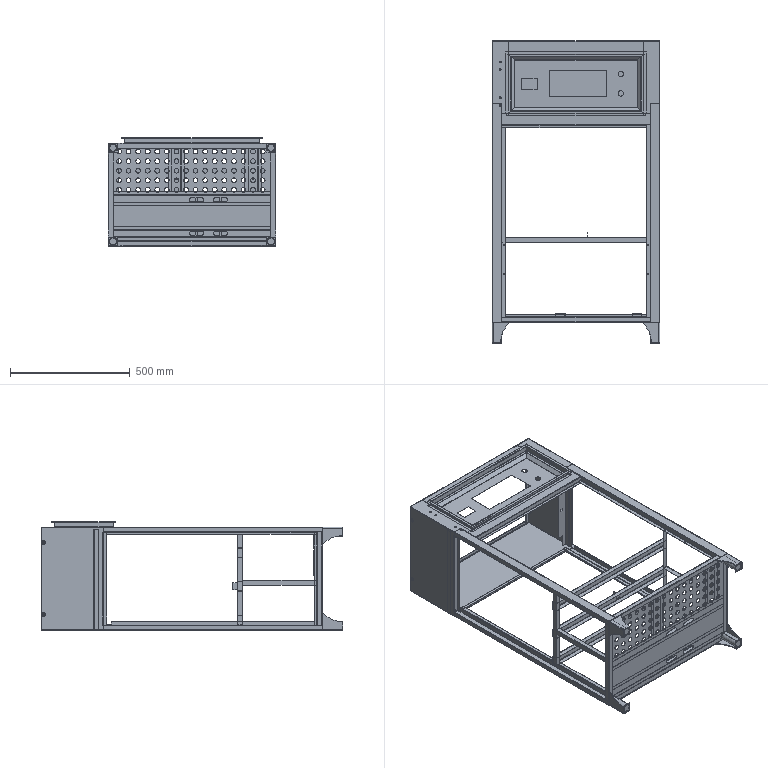Assembly | SolidWorks | mm | 51 component files | 51 solids | 1512 faces | box 700 x 1261 x 452 mm | volume 2289433 mm3 | plane 968 | cylinder 496 | cone 32 | spline 16 | commonest cylinder face diameters 20 x160 1.473 x95 3.473 x91 5 x48 6 x30 18 x12 10 x12 8 x8
Bill of materials:
12x1x12WeldedSquare | 4 | 304 | Thin, flat, square plate with no visible holes or other features.
CCQ-1.1-10Panel | 1 | 304 | Shallow rectangular tray or recessed panel. It has a flat floor, angled walls on all four sides, and a thin flat rim around the outside. The floor has one small rectangular cutout, one large rectangular cutout, and two small round holes.
CCQ-1.1-11UpperBeam1 | 1 | 304 | Long, thin-wall bent profile with a stepped, hat-like cross-section and rounded bends. In section it runs: bottom flange, vertical wall, raised horizontal wall, second vertical wall, short top return lip. One small round hole is near one end.
CCQ-1.1-12LowerBeam2 | 2 | 304 | Short, straight, thin-wall bent profile with three rounded bends. In section it runs: short leg, horizontal wall, long wall, horizontal wall. There is one small round hole near each end on one face.
CCQ-1.1-13UpperBeam2 | 1 | 304 | Long, thin-wall bent channel with three rounded bends. In section it has a short top lip, a vertical wall, a wide base, and a downward leg at the far edge. No holes are visible.
CCQ-1.1-14LowerSidePost1 | 2 | 304 | Long, thin-wall bent profile with five rounded bends. In section it forms a box-like channel with an outward flange on one side and an upward return lip on the other. No holes are visible.
CCQ-1.1-15LowerSidePost2 | 1 | 304 | Long, thin-wall bent profile with five rounded bends. In section it forms a near-closed box shape with two legs leaving in opposite directions (one horizontal flange, one vertical leg). There are small holes along one flange.
CCQ-1.1-16LowerSidePost3 | 1 | 304 | Long, thin-wall bent profile with five rounded bends. In section it forms a near-closed box shape with a downward leg and a horizontal outward flange. There is one round hole near one end on the top face and small holes along a flange. One flange is cut back near one end.
CCQ-1.1-17LowerBeam1 | 2 | 304 | Long bent profile with three rounded bends. In section it is an inverted U (channel) with an outward horizontal flange on one leg. The wall looks thicker relative to the section size than on the other profiles. No holes are visible.
CCQ-1.1-18Limiter | 1 | 304 | Short L-shaped angle with legs of about equal length and a single rounded bend. No holes are visible.
CCQ-1.1-19Support1 | 2 | 304 | Straight hat-section (omega-shaped) profile. It has a raised flat top, two vertical walls, and two outward flanges at the base, with rounded bends. There are two small round holes on the raised top face.
CCQ-1.1-1AngleIron | 2 | 304 | Long, slender L-shaped angle with legs of about equal length and a single rounded bend. No holes are visible.
CCQ-1.1-20Support2 | 2 | 304 | Long, straight hat-section (omega) profile made of thin formed sheet: a central U-shaped channel with two outward flanges, plus two obround slots through the channel floor.
CCQ-1.1-21SupportBendPart | 4 | 304 | Short thin angle piece with two legs at 90 degrees joined by a rounded bend. Each leg has a large concave curved cutout on its free edge, so the legs taper toward the bend corner.
CCQ-1.1-22VerticalAngleIron | 2 | 304 | Long, straight, plain L-angle profile of thin wall with a rounded inside bend and roughly equal legs.
CCQ-1.1-23BendPart | 3 | 304 | Long, straight C/U channel profile with a flat web, two parallel flanges and rounded bends. Two small round holes sit close together in the web near one end.
CCQ-1.1-2UpperAngleIron | 2 | 304 | Straight L-angle profile with unequal leg treatment: one leg runs the full length, while the other leg covers only a central portion, with stepped cutbacks at both ends. That partial leg has two elongated slots.
CCQ-1.1-3SideUpperPlate2 | 2 | 304 | Large, flat, rectangular thin sheet panel with formed edges. One long edge has a short return flange. The opposite edge has a flange with a small offset/downturned lip (joggle-like step). There are two small round holes near one side and a narrower, shorter flange strip along the other side.
CCQ-1.1-4SideUpperPlate1 | 1 | 304 | Rectangular, flat thin sheet panel with short upturned flanges along both long edges. One edge has an outward offset step before its lip. Small holes are visible near the flange ends.
CCQ-1.1-5SideUpperPlate3 | 1 | 304 | Elongated formed sheet bracket. A flat base plate joins a vertical wall that ends in a top return flange, giving a hook/C profile along one edge. A long rectangular slot runs through the vertical wall. The base plate outline has a stepped notch at one end, and the base plate extends past the formed channel at the other end.
CCQ-1.1-6SideUpperPlate4 | 1 | 304 | Elongated formed sheet bracket. A flat base plate joins a vertical wall with a top return flange (hook/C profile) along one edge. The flat plate has three round holes, and its outline has a stepped notch at one end. A short angled lip/flange sits at the other end.
CCQ-1.1-7BasePlate | 1 | 304 | Flat, thin rectangular plate with a regular perforation grid of 5 rows by 16 columns of round holes in its upper area. Below the grid are four obround slots in two horizontal pairs.
CCQ-1.1-8WeldedPlate | 4 | 304 | Rectangular plate/slab with significant thickness. It has a stepped (rabbet or tongue-like) edge feature along one side, where a slightly offset, shorter strip projects beyond the main face outline.
CCQ-1.1-9WeldedPipe | 4 | 304 | Plain straight cylindrical tube (hollow round section) with a uniform wall and square-cut open ends.
hex nuts, style 1-grades ab gb | 4 |  | Hexagonal prism with a central cylindrical through-bore and chamfered edges on both ends; general shape of a hex nut.
Mates:
1. coincident | CCQ-1.1-15LowerSidePost2-1 face at (0, 457.5, 20) dir (0, 0, 1) | CCQ-1.1-16LowerSidePost3-2 face at (-620, -457.5, 20) dir (0, 0, 1)
2. coincident | CCQ-1.1-15LowerSidePost2-1 face at (1, -457.5, 18.263) dir (0, -1, 0) | CCQ-1.1-16LowerSidePost3-2 face at (-659, -457.5, 18.263) dir (0, -1, 0)
3. distance | CCQ-1.1-15LowerSidePost2-1 face at (40, 457.5, 20) dir (1, 0, 0) | CCQ-1.1-16LowerSidePost3-2 face at (-660, -457.5, 20) dir (-1, 0, 0)
4. coincident | CCQ-1.1-15LowerSidePost2-1 face at (40, 457.5, 20) dir (1, 0, 0) | CCQ-1.1-14LowerSidePost1-3 face at (40, -457.5, -410) dir (1, 0, 0)
5. coincident | CCQ-1.1-14LowerSidePost1-3 face at (0, -457.5, -410) dir (0, 0, -1) | CCQ-1.1-14LowerSidePost1-4 face at (-620, 457.5, -410) dir (0, 0, -1)
6. coincident | CCQ-1.1-16LowerSidePost3-2 face at (-660, -457.5, 20) dir (-1, 0, 0) | CCQ-1.1-14LowerSidePost1-4 face at (-660, 457.5, -410) dir (-1, 0, 0)
7. coincident | CCQ-1.1-16LowerSidePost3-2 face at (-621, 457.5, 18.263) dir (0, 1, 0) | CCQ-1.1-14LowerSidePost1-4 face at (-659, 457.5, -408.263) dir (0, 1, 0)
8. coincident | CCQ-1.1-16LowerSidePost3-2 face at (-620, -457.5, 20) dir (0, 0, 1) | CCQ-1.1-17LowerBeam1-1 face at (0, -456.5, 20) dir (0, 0, 1)
9. coincident | CCQ-1.1-16LowerSidePost3-2 face at (-620, -457.5, -2) dir (1, 0, 0) | CCQ-1.1-17LowerBeam1-1 face at (-620, -437.237, 20) dir (-1, 0, 0)
10. coincident | CCQ-1.1-14LowerSidePost1-4 face at (-620, 457.5, -410) dir (0, 0, -1) | CCQ-1.1-17LowerBeam1-2 face at (-620, -456.5, -410) dir (0, 0, -1)
11. coincident | CCQ-1.1-14LowerSidePost1-4 face at (-620, 457.5, -388) dir (1, 0, 0) | CCQ-1.1-17LowerBeam1-2 face at (-620, -434.763, -388) dir (-1, 0, 0)
12. coincident | CCQ-1.1-14LowerSidePost1-4 face at (-621, -457.5, -408.263) dir (0, -1, 0) | CCQ-1.1-17LowerBeam1-2 face at (-620, -457.5, -409) dir (0, -1, 0)
13. coincident | CCQ-1.1-14LowerSidePost1-4 face at (-660, 457.5, -390) dir (0, 0, 1) | CCQ-1.1-12LowerBeam2-1 face at (-660, -437.237, -390) dir (0, 0, -1)
14. coincident | CCQ-1.1-14LowerSidePost1-4 face at (-660, 457.5, -410) dir (-1, 0, 0) | CCQ-1.1-12LowerBeam2-1 face at (-660, -456.5, 0) dir (-1, 0, 0)
15. coincident | CCQ-1.1-14LowerSidePost1-4 face at (-659, -457.5, -391.737) dir (0, -1, 0) | CCQ-1.1-12LowerBeam2-1 face at (-659, -457.5, 0) dir (0, -1, 0)
16. coincident | CCQ-1.1-15LowerSidePost2-1 face at (40, 457.5, 0) dir (0, 0, -1) | CCQ-1.1-12LowerBeam2-2 face at (38.263, -455.763, 0) dir (0, 0, 1)
17. coincident | CCQ-1.1-15LowerSidePost2-1 face at (40, 457.5, 20) dir (1, 0, 0) | CCQ-1.1-12LowerBeam2-2 face at (40, -456.5, -390) dir (1, 0, 0)
18. coincident | CCQ-1.1-17LowerBeam1-1 face at (0, -457.5, 19) dir (0, -1, 0) | CCQ-1.1-12LowerBeam2-2 face at (39, -457.5, -390) dir (0, -1, 0)
19. coincident | CCQ-1.1-12LowerBeam2-2 face at (39, -457.5, -390) dir (0, -1, 0) | CCQ-1.1-7BasePlate-1 face at (-310, -457.5, -195) dir (0, 1, 0)
20. coincident | CCQ-1.1-14LowerSidePost1-3 face at (0, -457.5, -410) dir (0, 0, -1) | CCQ-1.1-7BasePlate-1 face at (-660, -457.5, -410) dir (0, 0, -1)
21. coincident | CCQ-1.1-14LowerSidePost1-3 face at (40, -457.5, -410) dir (1, 0, 0) | CCQ-1.1-7BasePlate-1 face at (40, -457.5, 20) dir (1, 0, 0)
22. coincident | CCQ-1.1-16LowerSidePost3-2 face at (-620, -457.5, 20) dir (0, 0, 1) | CCQ-1.1-11UpperBeam1-1 face at (0, 416.5, 20) dir (0, 0, 1)
23. coincident | CCQ-1.1-16LowerSidePost3-2 face at (-620, -457.5, -2) dir (1, 0, 0) | CCQ-1.1-11UpperBeam1-1 face at (-620, 366.5, 18.263) dir (-1, 0, 0)
24. coincident | CCQ-1.1-7BasePlate-1 face at (-310, -458.5, -195) dir (0, -1, 0) | CCQ-1.1-21SupportBendPart-1 face at (36.263, -458.5, 20) dir (0, 1, 0)
25. coincident | CCQ-1.1-12LowerBeam2-2 face at (40, -456.5, -390) dir (1, 0, 0) | CCQ-1.1-21SupportBendPart-1 face at (40, -458.5, 17) dir (1, 0, 0)
26. coincident | CCQ-1.1-17LowerBeam1-1 face at (0, -456.5, 20) dir (0, 0, 1) | CCQ-1.1-21SupportBendPart-1 face at (37, -458.5, 20) dir (0, 0, 1)
27. coincident | CCQ-1.1-21SupportBendPart-1 face at (37, -458.5, 17) dir (0, 0, -1) | CCQ-1.1-8WeldedPlate-3 face at (3, -543.5, 17) dir (0, 0, 1)
28. coincident | CCQ-1.1-21SupportBendPart-1 face at (37, -458.5, 17) dir (-1, 0, 0) | CCQ-1.1-8WeldedPlate-3 face at (37, -543.5, -17) dir (1, 0, 0)
29. coincident | CCQ-1.1-21SupportBendPart-1 face at (40, -543.5, 16.263) dir (0, -1, 0) | CCQ-1.1-8WeldedPlate-3 face at (20, -543.5, 0) dir (0, -1, 0)
30. coincident | CCQ-1.1-14LowerSidePost1-3 face at (0, -457.5, -410) dir (0, 0, -1) | CCQ-1.1-21SupportBendPart-2 face at (37, -458.5, -410) dir (0, 0, -1)
31. coincident | CCQ-1.1-12LowerBeam2-2 face at (40, -456.5, -390) dir (1, 0, 0) | CCQ-1.1-21SupportBendPart-2 face at (40, -458.5, -407) dir (1, 0, 0)
32. coincident | CCQ-1.1-7BasePlate-1 face at (-310, -458.5, -195) dir (0, -1, 0) | CCQ-1.1-21SupportBendPart-2 face at (36.263, -458.5, -406.263) dir (0, 1, 0)
33. coincident | CCQ-1.1-21SupportBendPart-2 face at (37, -458.5, -407) dir (0, 0, 1) | CCQ-1.1-8WeldedPlate-2 face at (3, -543.5, -407) dir (0, 0, -1)
34. coincident | CCQ-1.1-21SupportBendPart-2 face at (37, -458.5, -407) dir (-1, 0, 0) | CCQ-1.1-8WeldedPlate-2 face at (37, -543.5, -407) dir (1, 0, 0)
35. coincident | CCQ-1.1-21SupportBendPart-2 face at (36.263, -543.5, -410) dir (0, -1, 0) | CCQ-1.1-8WeldedPlate-2 face at (20, -543.5, -390) dir (0, -1, 0)
36. width | CCQ-1.1-4SideUpperPlate1-3 face at (40, 457.5, -409) dir (1, 0, 0) | CCQ-1.1-4SideUpperPlate1-3 face at (-660, 457.5, -410) dir (-1, 0, 0) | CCQ-1.1-12LowerBeam2-1 face at (-660, -456.5, 0) dir (-1, 0, 0) | CCQ-1.1-12LowerBeam2-2 face at (40, -456.5, -390) dir (1, 0, 0)
37. parallel | CCQ-1.1-7BasePlate-1 face at (-310, -457.5, -195) dir (0, 1, 0) | CCQ-1.1-4SideUpperPlate1-3 face at (-310, 717.5, -195) dir (0, 1, 0)
38. coincident | CCQ-1.1-14LowerSidePost1-3 face at (0, -457.5, -410) dir (0, 0, -1) | CCQ-1.1-4SideUpperPlate1-3 face at (-660, 457.5, -410) dir (0, 0, -1)
39. coincident | CCQ-1.1-14LowerSidePost1-4 face at (-659, 457.5, -408.263) dir (0, 1, 0) | CCQ-1.1-4SideUpperPlate1-3 face at (-310, 457.5, -195) dir (0, -1, 0)
40. coincident | CCQ-1.1-14LowerSidePost1-4 face at (-658.263, 457.5, -391) dir (0, 1, 0) | CCQ-1.1-3SideUpperPlate2-1 face at (-660, 457.5, -195) dir (0, -1, 0)
41. coincident | CCQ-1.1-14LowerSidePost1-4 face at (-660, 457.5, -410) dir (-1, 0, 0) | CCQ-1.1-3SideUpperPlate2-1 face at (-660, 717.5, 19) dir (-1, 0, 0)
42. coincident | CCQ-1.1-4SideUpperPlate1-3 face at (-660, 457.5, -409) dir (0, 0, 1) | CCQ-1.1-3SideUpperPlate2-1 face at (-658.263, 716.5, -409) dir (0, 0, -1)
43. coincident | CCQ-1.1-15LowerSidePost2-1 face at (38.263, 457.5, 1) dir (0, 1, 0) | CCQ-1.1-3SideUpperPlate2-2 face at (40, 457.5, -195) dir (0, -1, 0)
44. coincident | CCQ-1.1-15LowerSidePost2-1 face at (40, 457.5, 20) dir (1, 0, 0) | CCQ-1.1-3SideUpperPlate2-2 face at (40, 717.5, -409) dir (1, 0, 0)
45. coincident | CCQ-1.1-4SideUpperPlate1-3 face at (-660, 457.5, -409) dir (0, 0, 1) | CCQ-1.1-3SideUpperPlate2-2 face at (38.263, 715.763, -409) dir (0, 0, -1)
46. coincident | CCQ-1.1-16LowerSidePost3-2 face at (-621, 457.5, 18.263) dir (0, 1, 0) | CCQ-1.1-6SideUpperPlate4-1 face at (-620, 457.5, 20) dir (0, -1, 0)
47. coincident | CCQ-1.1-16LowerSidePost3-2 face at (-620, -457.5, 20) dir (0, 0, 1) | CCQ-1.1-6SideUpperPlate4-1 face at (-625.25, 567, 20) dir (0, 0, 1)
48. coincident | CCQ-1.1-3SideUpperPlate2-1 face at (-660, 717.5, 19) dir (-1, 0, 0) | CCQ-1.1-6SideUpperPlate4-1 face at (-660, 457.5, 20) dir (-1, 0, 0)
49. coincident | CCQ-1.1-6SideUpperPlate4-1 face at (-625.25, 567, 20) dir (0, 0, 1) | CCQ-1.1-5SideUpperPlate3-2 face at (5.25, 567, 20) dir (0, 0, 1)
50. coincident | CCQ-1.1-13UpperBeam2-1 face at (-310, 717.5, 19) dir (0, 1, 0) | CCQ-1.1-5SideUpperPlate3-2 face at (5.25, 717.5, 20) dir (0, 1, 0)
51. coincident | CCQ-1.1-13UpperBeam2-1 face at (-29.5, 662.5, 20) dir (1, 0, 0) | CCQ-1.1-5SideUpperPlate3-2 face at (-29.5, 567, 20) dir (-1, 0, 0)
52. coincident | CCQ-1.1-11UpperBeam1-1 face at (0, 416.5, 20) dir (0, 1, 0) | CCQ-1.1-5SideUpperPlate3-2 face at (-29.5, 416.5, 19) dir (0, -1, 0)
53. coincident | CCQ-1.1-7BasePlate-1 face at (-310, -458.5, -195) dir (0, -1, 0) | CCQ-1.1-9WeldedPipe-1 face at (20, -458.5, 0) dir (0, 1, 0)
54. tangent | CCQ-1.1-21SupportBendPart-1 face at (37, -458.5, 17) dir (0, 0, -1) | CCQ-1.1-9WeldedPipe-1 face at (20, -540.5, 0) dir (0, 1, 0) r 17
55. tangent | CCQ-1.1-21SupportBendPart-1 face at (37, -458.5, 17) dir (-1, 0, 0) | CCQ-1.1-9WeldedPipe-1 face at (20, -540.5, 0) dir (0, 1, 0) r 17
56. tangent | CCQ-1.1-21SupportBendPart-2 face at (37, -458.5, -407) dir (-1, 0, 0) | CCQ-1.1-9WeldedPipe-2 face at (20, -540.5, -390) dir (0, 1, 0) r 17
57. coincident | CCQ-1.1-7BasePlate-1 face at (-310, -458.5, -195) dir (0, -1, 0) | CCQ-1.1-9WeldedPipe-2 face at (20, -458.5, -390) dir (0, 1, 0)
58. tangent | CCQ-1.1-21SupportBendPart-2 face at (37, -458.5, -407) dir (0, 0, 1) | CCQ-1.1-9WeldedPipe-2 face at (20, -540.5, -390) dir (0, 1, 0) r 17
59. coincident | CCQ-1.1-3SideUpperPlate2-1 face at (-658.263, 715.763, 19) dir (0, 0, 1) | CCQ-1.1-6SideUpperPlate4-1 face at (-625.25, 567, 19) dir (0, 0, -1)
60. coincident | CCQ-1.1-11UpperBeam1-1 face at (0, 365.763, 0.7366) dir (1, 0, 0) | CCQ-1.1-5SideUpperPlate3-2 face at (0, 416.5, 19) dir (1, 0, 0)
61. coincident | CCQ-1.1-15LowerSidePost2-1 face at (39, 457.5, 18.263) dir (0, 1, 0) | CCQ-1.1-5SideUpperPlate3-2 face at (0, 457.5, 19) dir (0, -1, 0)
62. coincident | CCQ-1.1-13UpperBeam2-1 face at (-29.5, 715.763, 20) dir (0, 0, 1) | CCQ-1.1-6SideUpperPlate4-1 face at (-625.25, 567, 20) dir (0, 0, 1)
63. coincident | CCQ-1.1-7BasePlate-1 face at (-310, -457.5, -195) dir (0, 1, 0) | CCQ-1.1-19Support1-1 face at (-35, -457.5, -2) dir (0, -1, 0)
64. coincident | CCQ-1.1-7BasePlate-1 face at (-310, -457.5, -195) dir (0, 1, 0) | CCQ-1.1-20Support2-1 face at (19, -457.5, -327) dir (0, -1, 0)
65. parallel | CCQ-1.1-17LowerBeam1-2 face at (-620, -436.5, -387) dir (0, 0, 1) | CCQ-1.1-20Support2-1 face at (19, -436.5, -372) dir (0, 0, -1)
66. width | CCQ-1.1-20Support2-1 face at (19, -438.237, -343) dir (1, 0, 0) | CCQ-1.1-20Support2-1 face at (-639, -437.5, -343.737) dir (-1, 0, 0) | CCQ-1.1-12LowerBeam2-1 face at (-660, -456.5, 0) dir (-1, 0, 0) | CCQ-1.1-12LowerBeam2-2 face at (40, -456.5, -390) dir (1, 0, 0)
67. coincident | CCQ-1.1-19Support1-1 face at (-34.263, -455.763, -182) dir (0, 0, -1) | CCQ-1.1-20Support2-2 face at (19, -457.5, -182) dir (0, 0, 1)
68. coincident | CCQ-1.1-14LowerSidePost1-3 face at (-15, -457.5, -387) dir (0, 0, 1) | CCQ-1.1-1AngleIron-1 face at (15.263, -122.763, -387) dir (0, 0, -1)
69. coincident | CCQ-1.1-14LowerSidePost1-3 face at (17, -457.5, -390) dir (-1, 0, 0) | CCQ-1.1-1AngleIron-1 face at (17, -104.5, -387) dir (1, 0, 0)
70. distance | CCQ-1.1-7BasePlate-1 face at (-310, -458.5, -195) dir (0, -1, 0) | CCQ-1.1-1AngleIron-1 face at (17, -123.5, -387) dir (0, 1, 0)
71. coincident | CCQ-1.1-14LowerSidePost1-4 face at (-605, 457.5, -387) dir (0, 0, 1) | CCQ-1.1-1AngleIron-2 face at (-636, -122.763, -387) dir (0, 0, -1)
72. coincident | CCQ-1.1-14LowerSidePost1-4 face at (-637, 457.5, -390) dir (1, 0, 0) | CCQ-1.1-1AngleIron-2 face at (-637, -104.5, -2) dir (-1, 0, 0)
73. coincident | CCQ-1.1-1AngleIron-1 face at (17, -123.5, -387) dir (0, 1, 0) | CCQ-1.1-1AngleIron-2 face at (-637, -123.5, -2) dir (0, 1, 0)
74. width | CCQ-1.1-23BendPart-1 face at (-637.5, -105.237, -386) dir (-1, 0, 0) | CCQ-1.1-23BendPart-1 face at (17.5, -105.237, -348) dir (1, 0, 0) | CCQ-1.1-1AngleIron-1 face at (16, -104.5, -387) dir (-1, 0, 0) | CCQ-1.1-1AngleIron-2 face at (-636, -104.5, -2) dir (1, 0, 0)
75. coincident | CCQ-1.1-1AngleIron-1 face at (17, -123.5, -387) dir (0, 1, 0) | CCQ-1.1-23BendPart-1 face at (-637.5, -123.5, -386) dir (0, -1, 0)
76. coincident | CCQ-1.1-14LowerSidePost1-3 face at (-15, -457.5, -387) dir (0, 0, 1) | CCQ-1.1-23BendPart-1 face at (-637.5, -123.5, -387) dir (0, 0, -1)
77. coincident | CCQ-1.1-3SideUpperPlate2-1 face at (-659, 717.5, 19) dir (1, 0, 0) | CCQ-1.1-2UpperAngleIron-1 face at (-659, 497.5, -409) dir (-1, 0, 0)
78. coincident | CCQ-1.1-3SideUpperPlate2-1 face at (-659, 717.5, 19) dir (1, 0, 0) | CCQ-1.1-2UpperAngleIron-1 face at (-659, 497.5, -409) dir (-1, 0, 0)
79. coincident | CCQ-1.1-3SideUpperPlate2-2 face at (39, 717.5, -409) dir (-1, 0, 0) | CCQ-1.1-2UpperAngleIron-2 face at (39, 497.5, 11) dir (1, 0, 0)
80. coincident | CCQ-1.1-2UpperAngleIron-1 face at (-619, 497.5, -409) dir (0, 1, 0) | CCQ-1.1-2UpperAngleIron-2 face at (-1, 497.5, 11) dir (0, 1, 0)
81. coincident | CCQ-1.1-2UpperAngleIron-1 face at (-639, 487.5, -359) dir (0, 0, -1) | CCQ-1.1-2UpperAngleIron-2 face at (19, 487.5, -359) dir (0, 0, -1)
82. distance | CCQ-1.1-2UpperAngleIron-1 face at (-619, 496.5, -409) dir (0, -1, 0) | CCQ-1.1-23BendPart-1 face at (-637.5, -103.5, -387) dir (0, 1, 0)
83. width | CCQ-1.1-10Panel-1 face at (-38.574, -2136.368, 17.784) dir (0.7071, 0, -0.7071) | CCQ-1.1-10Panel-1 face at (-581.426, 3213.632, 17.784) dir (-0.7071, 0, -0.7071) | CCQ-1.1-5SideUpperPlate3-2 face at (-29.5, 567, 20) dir (-1, 0, 0) | CCQ-1.1-6SideUpperPlate4-1 face at (-590.5, 567, 19) dir (1, 0, 0)
84. width | CCQ-1.1-10Panel-1 face at (-3142.5, 424.705, 17.784) dir (0, -0.7071, -0.7071) | CCQ-1.1-10Panel-1 face at (2522.5, 652.558, 17.784) dir (0, 0.7071, -0.7071) | CCQ-1.1-11UpperBeam1-1 face at (-310, 416.5, 19) dir (0, 1, 0) | CCQ-1.1-13UpperBeam2-1 face at (-29.5, 660.763, 19) dir (0, -1, 0)
85. parallel | CCQ-1.1-13UpperBeam2-1 face at (-310, 717.5, 19) dir (0, 1, 0) | CCQ-1.1-10Panel-1 face at (2522.5, 672.774, 18) dir (0, 1, 0)
86. coincident | CCQ-1.1-6SideUpperPlate4-1 face at (-625.25, 567, 19) dir (0, 0, -1) | CCQ-1.1-10Panel-1 face at (2522.5, 652.774, 19) dir (0, 0, 1)
87. coincident | CCQ-1.1-23BendPart-2 face at (-637.5, -103.5, -247) dir (0, 1, 0) | CCQ-1.1-18Limiter-2 face at (-261, -103.5, -242) dir (0, -1, 0)
88. width | CCQ-1.1-18Limiter-2 face at (-260, -101.763, -242) dir (0, 0, -1) | CCQ-1.1-18Limiter-2 face at (-259.263, -101.763, -212) dir (0, 0, 1) | CCQ-1.1-23BendPart-2 face at (-637.5, -103.5, -207) dir (0, 0, 1) | CCQ-1.1-23BendPart-2 face at (-637.5, -123.5, -247) dir (0, 0, -1)
89. distance | CCQ-1.1-18Limiter-2 face at (-261, -83.5, -242) dir (-1, 0, 0) | CCQ-1.1-16LowerSidePost3-2 face at (-639, -457.5, 0) dir (1, 0, 0)
90. coincident | CCQ-1.1-4SideUpperPlate1-3 face at (-660, 457.5, -409) dir (0, 0, 1) | CCQ-1.1-2UpperAngleIron-1 edge at (-639, 497.5, -409) dir (-1, 0, 0)
91. coincident | CCQ-1.1-20Support2-2 face at (19, -436.5, -197) dir (0, 1, 0) | CCQ-1.1-22VerticalAngleIron-1 face at (15.263, -436.5, -203.737) dir (0, -1, 0)
92. coincident | CCQ-1.1-1AngleIron-1 face at (17, -104.5, -387) dir (1, 0, 0) | CCQ-1.1-22VerticalAngleIron-1 face at (17, -124.5, -202) dir (1, 0, 0)
93. distance | CCQ-1.1-22VerticalAngleIron-1 face at (-3, -124.5, -202) dir (0, 0, 1) | CCQ-1.1-20Support2-2 face at (19, -456.5, -197) dir (0, 0, 1)
94. coincident | CCQ-1.1-15LowerSidePost2-1 face at (1, -457.5, 18.263) dir (0, -1, 0) | CCQ-1.1-7BasePlate-1 face at (-310, -457.5, -195) dir (0, 1, 0)
95. width | CCQ-1.1-19Support1-1 face at (-35, -421.5, -2) dir (1, 0, 0) | CCQ-1.1-19Support1-1 face at (-75, -456.5, -2) dir (-1, 0, 0) | CCQ-1.1-7BasePlate-1 face at (-55, -448.5, -95) dir (0, -1, 0) r 10
96. parallel | CCQ-1.1-12LowerBeam2-2 face at (40, -456.5, -390) dir (1, 0, 0) | CCQ-1.1-19Support1-1 face at (-35, -421.5, -2) dir (1, 0, 0)
97. coincident | CCQ-1.1-3SideUpperPlate2-2 face at (39, 717.5, -409) dir (-1, 0, 0) | hex nuts, style 1-grades ab gb-5 face at (39, 707.5, -354.238) dir (1, 0, 0)
98. concentric | CCQ-1.1-3SideUpperPlate2-2 face at (30, 707.5, -345) dir (1, 0, 0) r 2.5 | hex nuts, style 1-grades ab gb-5 face at (30.6, 707.5, -345) dir (1, 0, 0) r 4.5
99. concentric | CCQ-1.1-3SideUpperPlate2-2 face at (30, 707.5, -45) dir (1, 0, 0) r 2.5 | hex nuts, style 1-grades ab gb-2 face at (30.6, 707.5, -45) dir (1, 0, 0) r 4.5
100. coincident | CCQ-1.1-3SideUpperPlate2-2 face at (39, 717.5, -409) dir (-1, 0, 0) | hex nuts, style 1-grades ab gb-2 face at (39, 707.5, -54.238) dir (1, 0, 0)
101. coincident | CCQ-1.1-14LowerSidePost1-4 face at (-605, 457.5, -387) dir (0, 0, 1) | CCQ-1.1-20Support2-1 face at (19, -456.5, -387) dir (0, 0, -1)
102. coincident | CCQ-1.1-7BasePlate-1 face at (-310, -458.5, -195) dir (0, -1, 0) | CCQ-1.1-21SupportBendPart-5 face at (-656.263, -458.5, -410) dir (0, 1, 0)
103. coincident | CCQ-1.1-12LowerBeam2-1 face at (-660, -456.5, 0) dir (-1, 0, 0) | CCQ-1.1-21SupportBendPart-5 face at (-660, -458.5, -407) dir (-1, 0, 0)
104. coincident | CCQ-1.1-17LowerBeam1-2 face at (-620, -456.5, -410) dir (0, 0, -1) | CCQ-1.1-21SupportBendPart-5 face at (-657, -458.5, -410) dir (0, 0, -1)
105. coincident | CCQ-1.1-12LowerBeam2-1 face at (-660, -456.5, 0) dir (-1, 0, 0) | CCQ-1.1-21SupportBendPart-6 face at (-660, -458.5, 17) dir (-1, 0, 0)
106. coincident | CCQ-1.1-17LowerBeam1-1 face at (0, -456.5, 20) dir (0, 0, 1) | CCQ-1.1-21SupportBendPart-6 face at (-657, -458.5, 20) dir (0, 0, 1)
107. coincident | CCQ-1.1-7BasePlate-1 face at (-310, -458.5, -195) dir (0, -1, 0) | CCQ-1.1-21SupportBendPart-6 face at (-656.263, -458.5, 16.263) dir (0, 1, 0)
108. coincident | CCQ-1.1-13UpperBeam2-1 face at (-29.5, 661.763, 40.263) dir (1, 0, 0) | 12x1x12WeldedSquare-1 face at (-29.5, 672.5, 41) dir (-1, 0, 0)
109. coincident | CCQ-1.1-5SideUpperPlate3-2 face at (5.25, 567, 42) dir (0, 0, 1) | 12x1x12WeldedSquare-1 face at (-23.5, 666.5, 42) dir (0, 0, 1)
110. coincident | CCQ-1.1-5SideUpperPlate3-2 face at (-17.5, 660.5, 42) dir (0, 1, 0) | 12x1x12WeldedSquare-1 face at (-29.5, 660.5, 41) dir (0, -1, 0)
111. coincident | CCQ-1.1-11UpperBeam1-1 face at (-30, 404.5, 42) dir (1, 0, 0) | 12x1x12WeldedSquare-2 face at (-30, 416.5, 41) dir (-1, 0, 0)
112. coincident | CCQ-1.1-5SideUpperPlate3-2 face at (-28.5, 416.5, 42) dir (0, -1, 0) | 12x1x12WeldedSquare-2 face at (-30, 416.5, 41) dir (0, 1, 0)
113. coincident | CCQ-1.1-11UpperBeam1-1 face at (-310, 367.5, 42) dir (0, 0, 1) | 12x1x12WeldedSquare-2 face at (-24, 410.5, 42) dir (0, 0, 1)